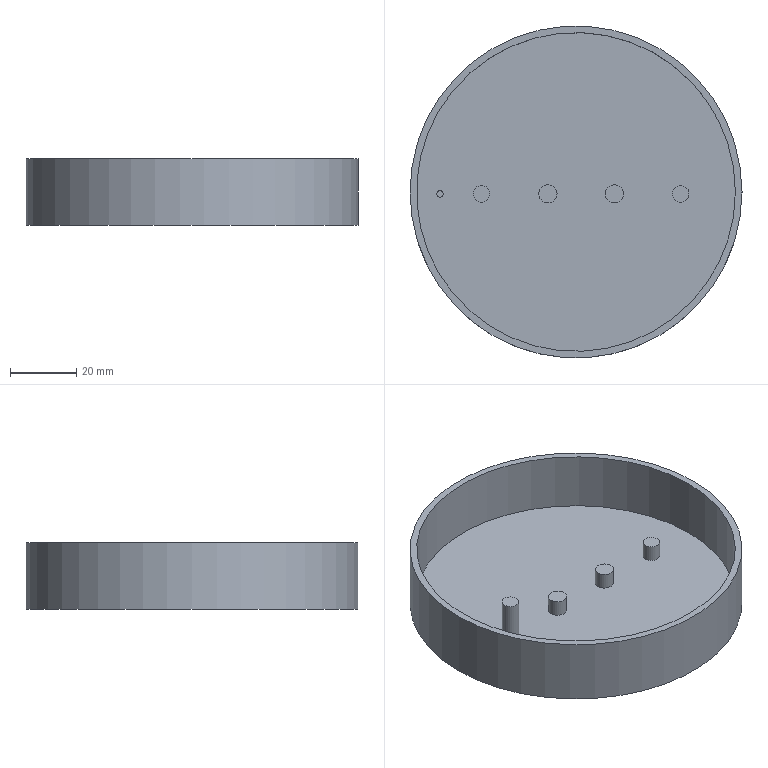Component | NX | BASE | 1 solid | 15 faces | box 100 x 100 x 20 mm | volume 27392 mm3 | plane 8 | cylinder 7 | commonest cylinder face diameters 5 x2 5.5 x2 100 x1 96 x1 2 x1
STEP:
#1=CARTESIAN_POINT('',(0.,0.,0.));
#2=DIRECTION('',(0.,0.,1.));
#3=DIRECTION('',(1.,0.,0.));
#4=AXIS2_PLACEMENT_3D('',#1,#2,#3);
#5=CARTESIAN_POINT('',(48.463,-15.037,-0.4905));
#6=VERTEX_POINT('',#5);
#7=CARTESIAN_POINT('',(-1.537,-15.037,-0.4905));
#8=DIRECTION('',(0.,0.,1.));
#9=DIRECTION('',(1.,0.,0.));
#10=AXIS2_PLACEMENT_3D('',#7,#8,#9);
#11=CIRCLE('',#10,50.);
#12=CARTESIAN_POINT('',(-1.537,-15.037,-0.4905));
#13=DIRECTION('',(0.,0.,-1.));
#14=DIRECTION('',(-1.,0.,0.));
#15=AXIS2_PLACEMENT_3D('',#12,#13,#14);
#16=CYLINDRICAL_SURFACE('',#15,50.);
#17=CARTESIAN_POINT('',(9.425,0.));
#18=DIRECTION('',(-1.,0.));
#19=VECTOR('',#18,1.);
#20=LINE('',#17,#19);
#21=(GEOMETRIC_REPRESENTATION_CONTEXT(2)PARAMETRIC_REPRESENTATION_CONTEXT()REPRESENTATION_CONTEXT('',''));
#22=DEFINITIONAL_REPRESENTATION('',(#20),#21);
#23=PCURVE('',#16,#22);
#24=CARTESIAN_POINT('',(-1.537,-15.037,-0.4905));
#25=DIRECTION('',(0.,0.,1.));
#26=DIRECTION('',(1.,0.,0.));
#27=AXIS2_PLACEMENT_3D('',#24,#25,#26);
#28=PLANE('',#27);
#29=CARTESIAN_POINT('',(0.,0.));
#30=DIRECTION('',(1.,0.));
#31=AXIS2_PLACEMENT_2D('',#29,#30);
#32=CIRCLE('',#31,50.);
#33=(GEOMETRIC_REPRESENTATION_CONTEXT(2)PARAMETRIC_REPRESENTATION_CONTEXT()REPRESENTATION_CONTEXT('',''));
#34=DEFINITIONAL_REPRESENTATION('',(#32),#33);
#35=PCURVE('',#28,#34);
#36=SURFACE_CURVE('',#11,(#23,#35),.PCURVE_S1.);
#37=EDGE_CURVE('',#6,#6,#36,.T.);
#38=ORIENTED_EDGE('',*,*,#37,.F.);
#39=CARTESIAN_POINT('',(48.463,-15.037,-20.49));
#40=VERTEX_POINT('',#39);
#41=CARTESIAN_POINT('',(48.463,-15.037,-0.4905));
#42=CARTESIAN_POINT('',(48.463,-15.037,-20.49));
#43=B_SPLINE_CURVE_WITH_KNOTS('',1,(#41,#42),.UNSPECIFIED.,.F.,.F.,(2,2),(0.,20.),.PIECEWISE_BEZIER_KNOTS.);
#44=CARTESIAN_POINT('',(9.425,0.));
#45=DIRECTION('',(0.,1.));
#46=VECTOR('',#45,1.);
#47=LINE('',#44,#46);
#48=(GEOMETRIC_REPRESENTATION_CONTEXT(2)PARAMETRIC_REPRESENTATION_CONTEXT()REPRESENTATION_CONTEXT('',''));
#49=DEFINITIONAL_REPRESENTATION('',(#47),#48);
#50=PCURVE('',#16,#49);
#51=CARTESIAN_POINT('',(3.142,0.));
#52=DIRECTION('',(0.,1.));
#53=VECTOR('',#52,1.);
#54=LINE('',#51,#53);
#55=(GEOMETRIC_REPRESENTATION_CONTEXT(2)PARAMETRIC_REPRESENTATION_CONTEXT()REPRESENTATION_CONTEXT('',''));
#56=DEFINITIONAL_REPRESENTATION('',(#54),#55);
#57=PCURVE('',#16,#56);
#58=SEAM_CURVE('',#43,(#50,#57),.PCURVE_S1.);
#59=EDGE_CURVE('',#6,#40,#58,.T.);
#60=ORIENTED_EDGE('',*,*,#59,.T.);
#61=CARTESIAN_POINT('',(-1.537,-15.037,-20.49));
#62=DIRECTION('',(0.,0.,1.));
#63=DIRECTION('',(1.,0.,0.));
#64=AXIS2_PLACEMENT_3D('',#61,#62,#63);
#65=CIRCLE('',#64,50.);
#66=CARTESIAN_POINT('',(9.425,20.));
#67=DIRECTION('',(-1.,0.));
#68=VECTOR('',#67,1.);
#69=LINE('',#66,#68);
#70=(GEOMETRIC_REPRESENTATION_CONTEXT(2)PARAMETRIC_REPRESENTATION_CONTEXT()REPRESENTATION_CONTEXT('',''));
#71=DEFINITIONAL_REPRESENTATION('',(#69),#70);
#72=PCURVE('',#16,#71);
#73=CARTESIAN_POINT('',(-1.537,-15.037,-20.49));
#74=DIRECTION('',(0.,0.,1.));
#75=DIRECTION('',(1.,0.,0.));
#76=AXIS2_PLACEMENT_3D('',#73,#74,#75);
#77=PLANE('',#76);
#78=CARTESIAN_POINT('',(0.,0.));
#79=DIRECTION('',(1.,0.));
#80=AXIS2_PLACEMENT_2D('',#78,#79);
#81=CIRCLE('',#80,50.);
#82=(GEOMETRIC_REPRESENTATION_CONTEXT(2)PARAMETRIC_REPRESENTATION_CONTEXT()REPRESENTATION_CONTEXT('',''));
#83=DEFINITIONAL_REPRESENTATION('',(#81),#82);
#84=PCURVE('',#77,#83);
#85=SURFACE_CURVE('',#65,(#72,#84),.PCURVE_S1.);
#86=EDGE_CURVE('',#40,#40,#85,.T.);
#87=ORIENTED_EDGE('',*,*,#86,.T.);
#88=ORIENTED_EDGE('',*,*,#59,.F.);
#89=EDGE_LOOP('',(#38,#60,#87,#88));
#90=FACE_BOUND('',#89,.T.);
#91=ADVANCED_FACE('',(#90),#16,.T.);
#92=CARTESIAN_POINT('',(46.463,-15.037,-0.4905));
#93=VERTEX_POINT('',#92);
#94=CARTESIAN_POINT('',(-1.537,-15.037,-0.4905));
#95=DIRECTION('',(0.,0.,1.));
#96=DIRECTION('',(1.,0.,0.));
#97=AXIS2_PLACEMENT_3D('',#94,#95,#96);
#98=CIRCLE('',#97,48.);
#99=CARTESIAN_POINT('',(0.,0.));
#100=DIRECTION('',(1.,0.));
#101=AXIS2_PLACEMENT_2D('',#99,#100);
#102=CIRCLE('',#101,48.);
#103=(GEOMETRIC_REPRESENTATION_CONTEXT(2)PARAMETRIC_REPRESENTATION_CONTEXT()REPRESENTATION_CONTEXT('',''));
#104=DEFINITIONAL_REPRESENTATION('',(#102),#103);
#105=PCURVE('',#28,#104);
#106=CARTESIAN_POINT('',(-1.537,-15.037,-0.4905));
#107=DIRECTION('',(0.,0.,-1.));
#108=DIRECTION('',(-1.,0.,0.));
#109=AXIS2_PLACEMENT_3D('',#106,#107,#108);
#110=CYLINDRICAL_SURFACE('',#109,48.);
#111=CARTESIAN_POINT('',(9.425,0.));
#112=DIRECTION('',(-1.,0.));
#113=VECTOR('',#112,1.);
#114=LINE('',#111,#113);
#115=(GEOMETRIC_REPRESENTATION_CONTEXT(2)PARAMETRIC_REPRESENTATION_CONTEXT()REPRESENTATION_CONTEXT('',''));
#116=DEFINITIONAL_REPRESENTATION('',(#114),#115);
#117=PCURVE('',#110,#116);
#118=SURFACE_CURVE('',#98,(#105,#117),.PCURVE_S1.);
#119=EDGE_CURVE('',#93,#93,#118,.T.);
#120=ORIENTED_EDGE('',*,*,#119,.F.);
#121=EDGE_LOOP('',(#120));
#122=FACE_BOUND('',#121,.T.);
#123=ORIENTED_EDGE('',*,*,#37,.T.);
#124=EDGE_LOOP('',(#123));
#125=FACE_BOUND('',#124,.T.);
#126=ADVANCED_FACE('',(#122,#125),#28,.T.);
#127=ORIENTED_EDGE('',*,*,#86,.F.);
#128=EDGE_LOOP('',(#127));
#129=FACE_BOUND('',#128,.T.);
#130=ADVANCED_FACE('',(#129),#77,.F.);
#131=ORIENTED_EDGE('',*,*,#119,.F.);
#132=CARTESIAN_POINT('',(46.463,-15.037,-18.49));
#133=VERTEX_POINT('',#132);
#134=CARTESIAN_POINT('',(46.463,-15.037,-0.4905));
#135=CARTESIAN_POINT('',(46.463,-15.037,-18.49));
#136=B_SPLINE_CURVE_WITH_KNOTS('',1,(#134,#135),.UNSPECIFIED.,.F.,.F.,(2,2),(0.,18.),.PIECEWISE_BEZIER_KNOTS.);
#137=CARTESIAN_POINT('',(9.425,0.));
#138=DIRECTION('',(0.,1.));
#139=VECTOR('',#138,1.);
#140=LINE('',#137,#139);
#141=(GEOMETRIC_REPRESENTATION_CONTEXT(2)PARAMETRIC_REPRESENTATION_CONTEXT()REPRESENTATION_CONTEXT('',''));
#142=DEFINITIONAL_REPRESENTATION('',(#140),#141);
#143=PCURVE('',#110,#142);
#144=CARTESIAN_POINT('',(3.142,0.));
#145=DIRECTION('',(0.,1.));
#146=VECTOR('',#145,1.);
#147=LINE('',#144,#146);
#148=(GEOMETRIC_REPRESENTATION_CONTEXT(2)PARAMETRIC_REPRESENTATION_CONTEXT()REPRESENTATION_CONTEXT('',''));
#149=DEFINITIONAL_REPRESENTATION('',(#147),#148);
#150=PCURVE('',#110,#149);
#151=SEAM_CURVE('',#136,(#143,#150),.PCURVE_S1.);
#152=EDGE_CURVE('',#93,#133,#151,.T.);
#153=ORIENTED_EDGE('',*,*,#152,.T.);
#154=CARTESIAN_POINT('',(-1.537,-15.037,-18.49));
#155=DIRECTION('',(0.,0.,1.));
#156=DIRECTION('',(1.,0.,0.));
#157=AXIS2_PLACEMENT_3D('',#154,#155,#156);
#158=CIRCLE('',#157,48.);
#159=CARTESIAN_POINT('',(9.425,18.));
#160=DIRECTION('',(-1.,0.));
#161=VECTOR('',#160,1.);
#162=LINE('',#159,#161);
#163=(GEOMETRIC_REPRESENTATION_CONTEXT(2)PARAMETRIC_REPRESENTATION_CONTEXT()REPRESENTATION_CONTEXT('',''));
#164=DEFINITIONAL_REPRESENTATION('',(#162),#163);
#165=PCURVE('',#110,#164);
#166=CARTESIAN_POINT('',(-1.537,-15.037,-18.49));
#167=DIRECTION('',(0.,0.,1.));
#168=DIRECTION('',(1.,0.,0.));
#169=AXIS2_PLACEMENT_3D('',#166,#167,#168);
#170=PLANE('',#169);
#171=CARTESIAN_POINT('',(0.,0.));
#172=DIRECTION('',(1.,0.));
#173=AXIS2_PLACEMENT_2D('',#171,#172);
#174=CIRCLE('',#173,48.);
#175=(GEOMETRIC_REPRESENTATION_CONTEXT(2)PARAMETRIC_REPRESENTATION_CONTEXT()REPRESENTATION_CONTEXT('',''));
#176=DEFINITIONAL_REPRESENTATION('',(#174),#175);
#177=PCURVE('',#170,#176);
#178=SURFACE_CURVE('',#158,(#165,#177),.PCURVE_S1.);
#179=EDGE_CURVE('',#133,#133,#178,.T.);
#180=ORIENTED_EDGE('',*,*,#179,.T.);
#181=ORIENTED_EDGE('',*,*,#152,.F.);
#182=EDGE_LOOP('',(#131,#153,#180,#181));
#183=FACE_BOUND('',#182,.F.);
#184=ADVANCED_FACE('',(#183),#110,.F.);
#185=CARTESIAN_POINT('',(-27.504,-15.585,-18.49));
#186=VERTEX_POINT('',#185);
#187=CARTESIAN_POINT('',(-30.004,-15.585,-18.49));
#188=DIRECTION('',(0.,0.,1.));
#189=DIRECTION('',(1.,0.,0.));
#190=AXIS2_PLACEMENT_3D('',#187,#188,#189);
#191=CIRCLE('',#190,2.5);
#192=CARTESIAN_POINT('',(-28.467,-0.5476));
#193=DIRECTION('',(1.,0.));
#194=AXIS2_PLACEMENT_2D('',#192,#193);
#195=CIRCLE('',#194,2.5);
#196=(GEOMETRIC_REPRESENTATION_CONTEXT(2)PARAMETRIC_REPRESENTATION_CONTEXT()REPRESENTATION_CONTEXT('',''));
#197=DEFINITIONAL_REPRESENTATION('',(#195),#196);
#198=PCURVE('',#170,#197);
#199=CARTESIAN_POINT('',(-30.004,-15.585,-18.49));
#200=DIRECTION('',(0.,0.,1.));
#201=DIRECTION('',(1.,0.,0.));
#202=AXIS2_PLACEMENT_3D('',#199,#200,#201);
#203=CYLINDRICAL_SURFACE('',#202,2.5);
#204=CARTESIAN_POINT('',(0.,0.));
#205=DIRECTION('',(1.,0.));
#206=VECTOR('',#205,1.);
#207=LINE('',#204,#206);
#208=(GEOMETRIC_REPRESENTATION_CONTEXT(2)PARAMETRIC_REPRESENTATION_CONTEXT()REPRESENTATION_CONTEXT('',''));
#209=DEFINITIONAL_REPRESENTATION('',(#207),#208);
#210=PCURVE('',#203,#209);
#211=SURFACE_CURVE('',#191,(#198,#210),.PCURVE_S1.);
#212=EDGE_CURVE('',#186,#186,#211,.T.);
#213=ORIENTED_EDGE('',*,*,#212,.F.);
#214=EDGE_LOOP('',(#213));
#215=FACE_BOUND('',#214,.T.);
#216=CARTESIAN_POINT('',(-7.254,-15.585,-18.49));
#217=VERTEX_POINT('',#216);
#218=CARTESIAN_POINT('',(-10.004,-15.585,-18.49));
#219=DIRECTION('',(0.,0.,1.));
#220=DIRECTION('',(1.,0.,0.));
#221=AXIS2_PLACEMENT_3D('',#218,#219,#220);
#222=CIRCLE('',#221,2.75);
#223=CARTESIAN_POINT('',(-8.467,-0.5476));
#224=DIRECTION('',(1.,0.));
#225=AXIS2_PLACEMENT_2D('',#223,#224);
#226=CIRCLE('',#225,2.75);
#227=(GEOMETRIC_REPRESENTATION_CONTEXT(2)PARAMETRIC_REPRESENTATION_CONTEXT()REPRESENTATION_CONTEXT('',''));
#228=DEFINITIONAL_REPRESENTATION('',(#226),#227);
#229=PCURVE('',#170,#228);
#230=CARTESIAN_POINT('',(-10.004,-15.585,-18.49));
#231=DIRECTION('',(0.,0.,1.));
#232=DIRECTION('',(1.,0.,0.));
#233=AXIS2_PLACEMENT_3D('',#230,#231,#232);
#234=CYLINDRICAL_SURFACE('',#233,2.75);
#235=CARTESIAN_POINT('',(0.,0.));
#236=DIRECTION('',(1.,0.));
#237=VECTOR('',#236,1.);
#238=LINE('',#235,#237);
#239=(GEOMETRIC_REPRESENTATION_CONTEXT(2)PARAMETRIC_REPRESENTATION_CONTEXT()REPRESENTATION_CONTEXT('',''));
#240=DEFINITIONAL_REPRESENTATION('',(#238),#239);
#241=PCURVE('',#234,#240);
#242=SURFACE_CURVE('',#222,(#229,#241),.PCURVE_S1.);
#243=EDGE_CURVE('',#217,#217,#242,.T.);
#244=ORIENTED_EDGE('',*,*,#243,.F.);
#245=EDGE_LOOP('',(#244));
#246=FACE_BOUND('',#245,.T.);
#247=CARTESIAN_POINT('',(12.746,-15.585,-18.49));
#248=VERTEX_POINT('',#247);
#249=CARTESIAN_POINT('',(9.996,-15.585,-18.49));
#250=DIRECTION('',(0.,0.,1.));
#251=DIRECTION('',(1.,0.,0.));
#252=AXIS2_PLACEMENT_3D('',#249,#250,#251);
#253=CIRCLE('',#252,2.75);
#254=CARTESIAN_POINT('',(11.533,-0.5476));
#255=DIRECTION('',(1.,0.));
#256=AXIS2_PLACEMENT_2D('',#254,#255);
#257=CIRCLE('',#256,2.75);
#258=(GEOMETRIC_REPRESENTATION_CONTEXT(2)PARAMETRIC_REPRESENTATION_CONTEXT()REPRESENTATION_CONTEXT('',''));
#259=DEFINITIONAL_REPRESENTATION('',(#257),#258);
#260=PCURVE('',#170,#259);
#261=CARTESIAN_POINT('',(9.996,-15.585,-18.49));
#262=DIRECTION('',(0.,0.,1.));
#263=DIRECTION('',(1.,0.,0.));
#264=AXIS2_PLACEMENT_3D('',#261,#262,#263);
#265=CYLINDRICAL_SURFACE('',#264,2.75);
#266=CARTESIAN_POINT('',(0.,0.));
#267=DIRECTION('',(1.,0.));
#268=VECTOR('',#267,1.);
#269=LINE('',#266,#268);
#270=(GEOMETRIC_REPRESENTATION_CONTEXT(2)PARAMETRIC_REPRESENTATION_CONTEXT()REPRESENTATION_CONTEXT('',''));
#271=DEFINITIONAL_REPRESENTATION('',(#269),#270);
#272=PCURVE('',#265,#271);
#273=SURFACE_CURVE('',#253,(#260,#272),.PCURVE_S1.);
#274=EDGE_CURVE('',#248,#248,#273,.T.);
#275=ORIENTED_EDGE('',*,*,#274,.F.);
#276=EDGE_LOOP('',(#275));
#277=FACE_BOUND('',#276,.T.);
#278=CARTESIAN_POINT('',(32.496,-15.585,-18.49));
#279=VERTEX_POINT('',#278);
#280=CARTESIAN_POINT('',(29.996,-15.585,-18.49));
#281=DIRECTION('',(0.,0.,1.));
#282=DIRECTION('',(1.,0.,0.));
#283=AXIS2_PLACEMENT_3D('',#280,#281,#282);
#284=CIRCLE('',#283,2.5);
#285=CARTESIAN_POINT('',(31.533,-0.5476));
#286=DIRECTION('',(1.,0.));
#287=AXIS2_PLACEMENT_2D('',#285,#286);
#288=CIRCLE('',#287,2.5);
#289=(GEOMETRIC_REPRESENTATION_CONTEXT(2)PARAMETRIC_REPRESENTATION_CONTEXT()REPRESENTATION_CONTEXT('',''));
#290=DEFINITIONAL_REPRESENTATION('',(#288),#289);
#291=PCURVE('',#170,#290);
#292=CARTESIAN_POINT('',(29.996,-15.585,-18.49));
#293=DIRECTION('',(0.,0.,1.));
#294=DIRECTION('',(1.,0.,0.));
#295=AXIS2_PLACEMENT_3D('',#292,#293,#294);
#296=CYLINDRICAL_SURFACE('',#295,2.5);
#297=CARTESIAN_POINT('',(0.,0.));
#298=DIRECTION('',(1.,0.));
#299=VECTOR('',#298,1.);
#300=LINE('',#297,#299);
#301=(GEOMETRIC_REPRESENTATION_CONTEXT(2)PARAMETRIC_REPRESENTATION_CONTEXT()REPRESENTATION_CONTEXT('',''));
#302=DEFINITIONAL_REPRESENTATION('',(#300),#301);
#303=PCURVE('',#296,#302);
#304=SURFACE_CURVE('',#284,(#291,#303),.PCURVE_S1.);
#305=EDGE_CURVE('',#279,#279,#304,.T.);
#306=ORIENTED_EDGE('',*,*,#305,.F.);
#307=EDGE_LOOP('',(#306));
#308=FACE_BOUND('',#307,.T.);
#309=CARTESIAN_POINT('',(-41.504,-15.585,-18.49));
#310=VERTEX_POINT('',#309);
#311=CARTESIAN_POINT('',(-42.504,-15.585,-18.49));
#312=DIRECTION('',(0.,0.,1.));
#313=DIRECTION('',(1.,0.,0.));
#314=AXIS2_PLACEMENT_3D('',#311,#312,#313);
#315=CIRCLE('',#314,1.);
#316=CARTESIAN_POINT('',(-40.967,-0.5476));
#317=DIRECTION('',(1.,0.));
#318=AXIS2_PLACEMENT_2D('',#316,#317);
#319=CIRCLE('',#318,1.);
#320=(GEOMETRIC_REPRESENTATION_CONTEXT(2)PARAMETRIC_REPRESENTATION_CONTEXT()REPRESENTATION_CONTEXT('',''));
#321=DEFINITIONAL_REPRESENTATION('',(#319),#320);
#322=PCURVE('',#170,#321);
#323=CARTESIAN_POINT('',(-42.504,-15.585,-15.49));
#324=DIRECTION('',(0.,0.,-1.));
#325=DIRECTION('',(-1.,0.,0.));
#326=AXIS2_PLACEMENT_3D('',#323,#324,#325);
#327=CYLINDRICAL_SURFACE('',#326,1.);
#328=CARTESIAN_POINT('',(9.425,3.));
#329=DIRECTION('',(-1.,0.));
#330=VECTOR('',#329,1.);
#331=LINE('',#328,#330);
#332=(GEOMETRIC_REPRESENTATION_CONTEXT(2)PARAMETRIC_REPRESENTATION_CONTEXT()REPRESENTATION_CONTEXT('',''));
#333=DEFINITIONAL_REPRESENTATION('',(#331),#332);
#334=PCURVE('',#327,#333);
#335=SURFACE_CURVE('',#315,(#322,#334),.PCURVE_S1.);
#336=EDGE_CURVE('',#310,#310,#335,.T.);
#337=ORIENTED_EDGE('',*,*,#336,.F.);
#338=EDGE_LOOP('',(#337));
#339=FACE_BOUND('',#338,.T.);
#340=ORIENTED_EDGE('',*,*,#179,.T.);
#341=EDGE_LOOP('',(#340));
#342=FACE_BOUND('',#341,.T.);
#343=ADVANCED_FACE('',(#215,#246,#277,#308,#339,#342),#170,.T.);
#344=CARTESIAN_POINT('',(-41.504,-15.585,-15.49));
#345=VERTEX_POINT('',#344);
#346=CARTESIAN_POINT('',(-42.504,-15.585,-15.49));
#347=DIRECTION('',(0.,0.,1.));
#348=DIRECTION('',(1.,0.,0.));
#349=AXIS2_PLACEMENT_3D('',#346,#347,#348);
#350=CIRCLE('',#349,1.);
#351=CARTESIAN_POINT('',(9.425,0.));
#352=DIRECTION('',(-1.,0.));
#353=VECTOR('',#352,1.);
#354=LINE('',#351,#353);
#355=(GEOMETRIC_REPRESENTATION_CONTEXT(2)PARAMETRIC_REPRESENTATION_CONTEXT()REPRESENTATION_CONTEXT('',''));
#356=DEFINITIONAL_REPRESENTATION('',(#354),#355);
#357=PCURVE('',#327,#356);
#358=CARTESIAN_POINT('',(-42.504,-15.585,-15.49));
#359=DIRECTION('',(0.,0.,1.));
#360=DIRECTION('',(1.,0.,0.));
#361=AXIS2_PLACEMENT_3D('',#358,#359,#360);
#362=PLANE('',#361);
#363=CARTESIAN_POINT('',(0.,0.));
#364=DIRECTION('',(1.,0.));
#365=AXIS2_PLACEMENT_2D('',#363,#364);
#366=CIRCLE('',#365,1.);
#367=(GEOMETRIC_REPRESENTATION_CONTEXT(2)PARAMETRIC_REPRESENTATION_CONTEXT()REPRESENTATION_CONTEXT('',''));
#368=DEFINITIONAL_REPRESENTATION('',(#366),#367);
#369=PCURVE('',#362,#368);
#370=SURFACE_CURVE('',#350,(#357,#369),.PCURVE_S1.);
#371=EDGE_CURVE('',#345,#345,#370,.T.);
#372=ORIENTED_EDGE('',*,*,#371,.F.);
#373=CARTESIAN_POINT('',(-41.504,-15.585,-15.49));
#374=CARTESIAN_POINT('',(-41.504,-15.585,-18.49));
#375=B_SPLINE_CURVE_WITH_KNOTS('',1,(#373,#374),.UNSPECIFIED.,.F.,.F.,(2,2),(0.,3.),.PIECEWISE_BEZIER_KNOTS.);
#376=CARTESIAN_POINT('',(9.425,0.));
#377=DIRECTION('',(0.,1.));
#378=VECTOR('',#377,1.);
#379=LINE('',#376,#378);
#380=(GEOMETRIC_REPRESENTATION_CONTEXT(2)PARAMETRIC_REPRESENTATION_CONTEXT()REPRESENTATION_CONTEXT('',''));
#381=DEFINITIONAL_REPRESENTATION('',(#379),#380);
#382=PCURVE('',#327,#381);
#383=CARTESIAN_POINT('',(3.142,0.));
#384=DIRECTION('',(0.,1.));
#385=VECTOR('',#384,1.);
#386=LINE('',#383,#385);
#387=(GEOMETRIC_REPRESENTATION_CONTEXT(2)PARAMETRIC_REPRESENTATION_CONTEXT()REPRESENTATION_CONTEXT('',''));
#388=DEFINITIONAL_REPRESENTATION('',(#386),#387);
#389=PCURVE('',#327,#388);
#390=SEAM_CURVE('',#375,(#382,#389),.PCURVE_S1.);
#391=EDGE_CURVE('',#345,#310,#390,.T.);
#392=ORIENTED_EDGE('',*,*,#391,.T.);
#393=ORIENTED_EDGE('',*,*,#336,.T.);
#394=ORIENTED_EDGE('',*,*,#391,.F.);
#395=EDGE_LOOP('',(#372,#392,#393,#394));
#396=FACE_BOUND('',#395,.T.);
#397=ADVANCED_FACE('',(#396),#327,.T.);
#398=ORIENTED_EDGE('',*,*,#371,.T.);
#399=EDGE_LOOP('',(#398));
#400=FACE_BOUND('',#399,.T.);
#401=ADVANCED_FACE('',(#400),#362,.T.);
#402=ORIENTED_EDGE('',*,*,#305,.T.);
#403=CARTESIAN_POINT('',(32.496,-15.585,-13.49));
#404=VERTEX_POINT('',#403);
#405=CARTESIAN_POINT('',(32.496,-15.585,-18.49));
#406=CARTESIAN_POINT('',(32.496,-15.585,-13.49));
#407=B_SPLINE_CURVE_WITH_KNOTS('',1,(#405,#406),.UNSPECIFIED.,.F.,.F.,(2,2),(0.,5.),.PIECEWISE_BEZIER_KNOTS.);
#408=CARTESIAN_POINT('',(6.283,0.));
#409=DIRECTION('',(0.,1.));
#410=VECTOR('',#409,1.);
#411=LINE('',#408,#410);
#412=(GEOMETRIC_REPRESENTATION_CONTEXT(2)PARAMETRIC_REPRESENTATION_CONTEXT()REPRESENTATION_CONTEXT('',''));
#413=DEFINITIONAL_REPRESENTATION('',(#411),#412);
#414=PCURVE('',#296,#413);
#415=CARTESIAN_POINT('',(0.,0.));
#416=DIRECTION('',(0.,1.));
#417=VECTOR('',#416,1.);
#418=LINE('',#415,#417);
#419=(GEOMETRIC_REPRESENTATION_CONTEXT(2)PARAMETRIC_REPRESENTATION_CONTEXT()REPRESENTATION_CONTEXT('',''));
#420=DEFINITIONAL_REPRESENTATION('',(#418),#419);
#421=PCURVE('',#296,#420);
#422=SEAM_CURVE('',#407,(#414,#421),.PCURVE_S1.);
#423=EDGE_CURVE('',#279,#404,#422,.T.);
#424=ORIENTED_EDGE('',*,*,#423,.T.);
#425=CARTESIAN_POINT('',(29.996,-15.585,-13.49));
#426=DIRECTION('',(0.,0.,1.));
#427=DIRECTION('',(1.,0.,0.));
#428=AXIS2_PLACEMENT_3D('',#425,#426,#427);
#429=CIRCLE('',#428,2.5);
#430=CARTESIAN_POINT('',(0.,5.));
#431=DIRECTION('',(1.,0.));
#432=VECTOR('',#431,1.);
#433=LINE('',#430,#432);
#434=(GEOMETRIC_REPRESENTATION_CONTEXT(2)PARAMETRIC_REPRESENTATION_CONTEXT()REPRESENTATION_CONTEXT('',''));
#435=DEFINITIONAL_REPRESENTATION('',(#433),#434);
#436=PCURVE('',#296,#435);
#437=CARTESIAN_POINT('',(29.996,-15.585,-13.49));
#438=DIRECTION('',(0.,0.,1.));
#439=DIRECTION('',(1.,0.,0.));
#440=AXIS2_PLACEMENT_3D('',#437,#438,#439);
#441=PLANE('',#440);
#442=CARTESIAN_POINT('',(0.,0.));
#443=DIRECTION('',(1.,0.));
#444=AXIS2_PLACEMENT_2D('',#442,#443);
#445=CIRCLE('',#444,2.5);
#446=(GEOMETRIC_REPRESENTATION_CONTEXT(2)PARAMETRIC_REPRESENTATION_CONTEXT()REPRESENTATION_CONTEXT('',''));
#447=DEFINITIONAL_REPRESENTATION('',(#445),#446);
#448=PCURVE('',#441,#447);
#449=SURFACE_CURVE('',#429,(#436,#448),.PCURVE_S1.);
#450=EDGE_CURVE('',#404,#404,#449,.T.);
#451=ORIENTED_EDGE('',*,*,#450,.F.);
#452=ORIENTED_EDGE('',*,*,#423,.F.);
#453=EDGE_LOOP('',(#402,#424,#451,#452));
#454=FACE_BOUND('',#453,.T.);
#455=ADVANCED_FACE('',(#454),#296,.T.);
#456=ORIENTED_EDGE('',*,*,#450,.T.);
#457=EDGE_LOOP('',(#456));
#458=FACE_BOUND('',#457,.T.);
#459=ADVANCED_FACE('',(#458),#441,.T.);
#460=ORIENTED_EDGE('',*,*,#274,.T.);
#461=CARTESIAN_POINT('',(12.746,-15.585,-13.49));
#462=VERTEX_POINT('',#461);
#463=CARTESIAN_POINT('',(12.746,-15.585,-18.49));
#464=CARTESIAN_POINT('',(12.746,-15.585,-13.49));
#465=B_SPLINE_CURVE_WITH_KNOTS('',1,(#463,#464),.UNSPECIFIED.,.F.,.F.,(2,2),(0.,5.),.PIECEWISE_BEZIER_KNOTS.);
#466=CARTESIAN_POINT('',(6.283,0.));
#467=DIRECTION('',(0.,1.));
#468=VECTOR('',#467,1.);
#469=LINE('',#466,#468);
#470=(GEOMETRIC_REPRESENTATION_CONTEXT(2)PARAMETRIC_REPRESENTATION_CONTEXT()REPRESENTATION_CONTEXT('',''));
#471=DEFINITIONAL_REPRESENTATION('',(#469),#470);
#472=PCURVE('',#265,#471);
#473=CARTESIAN_POINT('',(0.,0.));
#474=DIRECTION('',(0.,1.));
#475=VECTOR('',#474,1.);
#476=LINE('',#473,#475);
#477=(GEOMETRIC_REPRESENTATION_CONTEXT(2)PARAMETRIC_REPRESENTATION_CONTEXT()REPRESENTATION_CONTEXT('',''));
#478=DEFINITIONAL_REPRESENTATION('',(#476),#477);
#479=PCURVE('',#265,#478);
#480=SEAM_CURVE('',#465,(#472,#479),.PCURVE_S1.);
#481=EDGE_CURVE('',#248,#462,#480,.T.);
#482=ORIENTED_EDGE('',*,*,#481,.T.);
#483=CARTESIAN_POINT('',(9.996,-15.585,-13.49));
#484=DIRECTION('',(0.,0.,1.));
#485=DIRECTION('',(1.,0.,0.));
#486=AXIS2_PLACEMENT_3D('',#483,#484,#485);
#487=CIRCLE('',#486,2.75);
#488=CARTESIAN_POINT('',(0.,5.));
#489=DIRECTION('',(1.,0.));
#490=VECTOR('',#489,1.);
#491=LINE('',#488,#490);
#492=(GEOMETRIC_REPRESENTATION_CONTEXT(2)PARAMETRIC_REPRESENTATION_CONTEXT()REPRESENTATION_CONTEXT('',''));
#493=DEFINITIONAL_REPRESENTATION('',(#491),#492);
#494=PCURVE('',#265,#493);
#495=CARTESIAN_POINT('',(9.996,-15.585,-13.49));
#496=DIRECTION('',(0.,0.,1.));
#497=DIRECTION('',(1.,0.,0.));
#498=AXIS2_PLACEMENT_3D('',#495,#496,#497);
#499=PLANE('',#498);
#500=CARTESIAN_POINT('',(0.,0.));
#501=DIRECTION('',(1.,0.));
#502=AXIS2_PLACEMENT_2D('',#500,#501);
#503=CIRCLE('',#502,2.75);
#504=(GEOMETRIC_REPRESENTATION_CONTEXT(2)PARAMETRIC_REPRESENTATION_CONTEXT()REPRESENTATION_CONTEXT('',''));
#505=DEFINITIONAL_REPRESENTATION('',(#503),#504);
#506=PCURVE('',#499,#505);
#507=SURFACE_CURVE('',#487,(#494,#506),.PCURVE_S1.);
#508=EDGE_CURVE('',#462,#462,#507,.T.);
#509=ORIENTED_EDGE('',*,*,#508,.F.);
#510=ORIENTED_EDGE('',*,*,#481,.F.);
#511=EDGE_LOOP('',(#460,#482,#509,#510));
#512=FACE_BOUND('',#511,.T.);
#513=ADVANCED_FACE('',(#512),#265,.T.);
#514=ORIENTED_EDGE('',*,*,#508,.T.);
#515=EDGE_LOOP('',(#514));
#516=FACE_BOUND('',#515,.T.);
#517=ADVANCED_FACE('',(#516),#499,.T.);
#518=ORIENTED_EDGE('',*,*,#243,.T.);
#519=CARTESIAN_POINT('',(-7.254,-15.585,-13.49));
#520=VERTEX_POINT('',#519);
#521=CARTESIAN_POINT('',(-7.254,-15.585,-18.49));
#522=CARTESIAN_POINT('',(-7.254,-15.585,-13.49));
#523=B_SPLINE_CURVE_WITH_KNOTS('',1,(#521,#522),.UNSPECIFIED.,.F.,.F.,(2,2),(0.,5.),.PIECEWISE_BEZIER_KNOTS.);
#524=CARTESIAN_POINT('',(6.283,0.));
#525=DIRECTION('',(0.,1.));
#526=VECTOR('',#525,1.);
#527=LINE('',#524,#526);
#528=(GEOMETRIC_REPRESENTATION_CONTEXT(2)PARAMETRIC_REPRESENTATION_CONTEXT()REPRESENTATION_CONTEXT('',''));
#529=DEFINITIONAL_REPRESENTATION('',(#527),#528);
#530=PCURVE('',#234,#529);
#531=CARTESIAN_POINT('',(0.,0.));
#532=DIRECTION('',(0.,1.));
#533=VECTOR('',#532,1.);
#534=LINE('',#531,#533);
#535=(GEOMETRIC_REPRESENTATION_CONTEXT(2)PARAMETRIC_REPRESENTATION_CONTEXT()REPRESENTATION_CONTEXT('',''));
#536=DEFINITIONAL_REPRESENTATION('',(#534),#535);
#537=PCURVE('',#234,#536);
#538=SEAM_CURVE('',#523,(#530,#537),.PCURVE_S1.);
#539=EDGE_CURVE('',#217,#520,#538,.T.);
#540=ORIENTED_EDGE('',*,*,#539,.T.);
#541=CARTESIAN_POINT('',(-10.004,-15.585,-13.49));
#542=DIRECTION('',(0.,0.,1.));
#543=DIRECTION('',(1.,0.,0.));
#544=AXIS2_PLACEMENT_3D('',#541,#542,#543);
#545=CIRCLE('',#544,2.75);
#546=CARTESIAN_POINT('',(0.,5.));
#547=DIRECTION('',(1.,0.));
#548=VECTOR('',#547,1.);
#549=LINE('',#546,#548);
#550=(GEOMETRIC_REPRESENTATION_CONTEXT(2)PARAMETRIC_REPRESENTATION_CONTEXT()REPRESENTATION_CONTEXT('',''));
#551=DEFINITIONAL_REPRESENTATION('',(#549),#550);
#552=PCURVE('',#234,#551);
#553=CARTESIAN_POINT('',(-10.004,-15.585,-13.49));
#554=DIRECTION('',(0.,0.,1.));
#555=DIRECTION('',(1.,0.,0.));
#556=AXIS2_PLACEMENT_3D('',#553,#554,#555);
#557=PLANE('',#556);
#558=CARTESIAN_POINT('',(0.,0.));
#559=DIRECTION('',(1.,0.));
#560=AXIS2_PLACEMENT_2D('',#558,#559);
#561=CIRCLE('',#560,2.75);
#562=(GEOMETRIC_REPRESENTATION_CONTEXT(2)PARAMETRIC_REPRESENTATION_CONTEXT()REPRESENTATION_CONTEXT('',''));
#563=DEFINITIONAL_REPRESENTATION('',(#561),#562);
#564=PCURVE('',#557,#563);
#565=SURFACE_CURVE('',#545,(#552,#564),.PCURVE_S1.);
#566=EDGE_CURVE('',#520,#520,#565,.T.);
#567=ORIENTED_EDGE('',*,*,#566,.F.);
#568=ORIENTED_EDGE('',*,*,#539,.F.);
#569=EDGE_LOOP('',(#518,#540,#567,#568));
#570=FACE_BOUND('',#569,.T.);
#571=ADVANCED_FACE('',(#570),#234,.T.);
#572=ORIENTED_EDGE('',*,*,#566,.T.);
#573=EDGE_LOOP('',(#572));
#574=FACE_BOUND('',#573,.T.);
#575=ADVANCED_FACE('',(#574),#557,.T.);
#576=ORIENTED_EDGE('',*,*,#212,.T.);
#577=CARTESIAN_POINT('',(-27.504,-15.585,-5.49));
#578=VERTEX_POINT('',#577);
#579=CARTESIAN_POINT('',(-27.504,-15.585,-18.49));
#580=CARTESIAN_POINT('',(-27.504,-15.585,-5.49));
#581=B_SPLINE_CURVE_WITH_KNOTS('',1,(#579,#580),.UNSPECIFIED.,.F.,.F.,(2,2),(0.,13.),.PIECEWISE_BEZIER_KNOTS.);
#582=CARTESIAN_POINT('',(6.283,0.));
#583=DIRECTION('',(0.,1.));
#584=VECTOR('',#583,1.);
#585=LINE('',#582,#584);
#586=(GEOMETRIC_REPRESENTATION_CONTEXT(2)PARAMETRIC_REPRESENTATION_CONTEXT()REPRESENTATION_CONTEXT('',''));
#587=DEFINITIONAL_REPRESENTATION('',(#585),#586);
#588=PCURVE('',#203,#587);
#589=CARTESIAN_POINT('',(0.,0.));
#590=DIRECTION('',(0.,1.));
#591=VECTOR('',#590,1.);
#592=LINE('',#589,#591);
#593=(GEOMETRIC_REPRESENTATION_CONTEXT(2)PARAMETRIC_REPRESENTATION_CONTEXT()REPRESENTATION_CONTEXT('',''));
#594=DEFINITIONAL_REPRESENTATION('',(#592),#593);
#595=PCURVE('',#203,#594);
#596=SEAM_CURVE('',#581,(#588,#595),.PCURVE_S1.);
#597=EDGE_CURVE('',#186,#578,#596,.T.);
#598=ORIENTED_EDGE('',*,*,#597,.T.);
#599=CARTESIAN_POINT('',(-30.004,-15.585,-5.49));
#600=DIRECTION('',(0.,0.,1.));
#601=DIRECTION('',(1.,0.,0.));
#602=AXIS2_PLACEMENT_3D('',#599,#600,#601);
#603=CIRCLE('',#602,2.5);
#604=CARTESIAN_POINT('',(0.,13.));
#605=DIRECTION('',(1.,0.));
#606=VECTOR('',#605,1.);
#607=LINE('',#604,#606);
#608=(GEOMETRIC_REPRESENTATION_CONTEXT(2)PARAMETRIC_REPRESENTATION_CONTEXT()REPRESENTATION_CONTEXT('',''));
#609=DEFINITIONAL_REPRESENTATION('',(#607),#608);
#610=PCURVE('',#203,#609);
#611=CARTESIAN_POINT('',(-30.004,-15.585,-5.49));
#612=DIRECTION('',(0.,0.,1.));
#613=DIRECTION('',(1.,0.,0.));
#614=AXIS2_PLACEMENT_3D('',#611,#612,#613);
#615=PLANE('',#614);
#616=CARTESIAN_POINT('',(0.,0.));
#617=DIRECTION('',(1.,0.));
#618=AXIS2_PLACEMENT_2D('',#616,#617);
#619=CIRCLE('',#618,2.5);
#620=(GEOMETRIC_REPRESENTATION_CONTEXT(2)PARAMETRIC_REPRESENTATION_CONTEXT()REPRESENTATION_CONTEXT('',''));
#621=DEFINITIONAL_REPRESENTATION('',(#619),#620);
#622=PCURVE('',#615,#621);
#623=SURFACE_CURVE('',#603,(#610,#622),.PCURVE_S1.);
#624=EDGE_CURVE('',#578,#578,#623,.T.);
#625=ORIENTED_EDGE('',*,*,#624,.F.);
#626=ORIENTED_EDGE('',*,*,#597,.F.);
#627=EDGE_LOOP('',(#576,#598,#625,#626));
#628=FACE_BOUND('',#627,.T.);
#629=ADVANCED_FACE('',(#628),#203,.T.);
#630=ORIENTED_EDGE('',*,*,#624,.T.);
#631=EDGE_LOOP('',(#630));
#632=FACE_BOUND('',#631,.T.);
#633=ADVANCED_FACE('',(#632),#615,.T.);
#634=CLOSED_SHELL('',(#91,#126,#130,#184,#343,#397,#401,#455,#459,#513,#517,#571,#575,#629,#633));
#635=MANIFOLD_SOLID_BREP('',#634);
#636=(LENGTH_UNIT()NAMED_UNIT(*)SI_UNIT(.MILLI.,.METRE.));
#637=UNCERTAINTY_MEASURE_WITH_UNIT(LENGTH_MEASURE(0.00001),#636,'','');
#638=(NAMED_UNIT(*)PLANE_ANGLE_UNIT()SI_UNIT($,.RADIAN.));
#639=(NAMED_UNIT(*)SI_UNIT($,.STERADIAN.)SOLID_ANGLE_UNIT());
#640=(GEOMETRIC_REPRESENTATION_CONTEXT(3)GLOBAL_UNCERTAINTY_ASSIGNED_CONTEXT((#637))GLOBAL_UNIT_ASSIGNED_CONTEXT((#636,#638,#639))REPRESENTATION_CONTEXT('',''));
#641=ADVANCED_BREP_SHAPE_REPRESENTATION('',(#4,#635),#640);